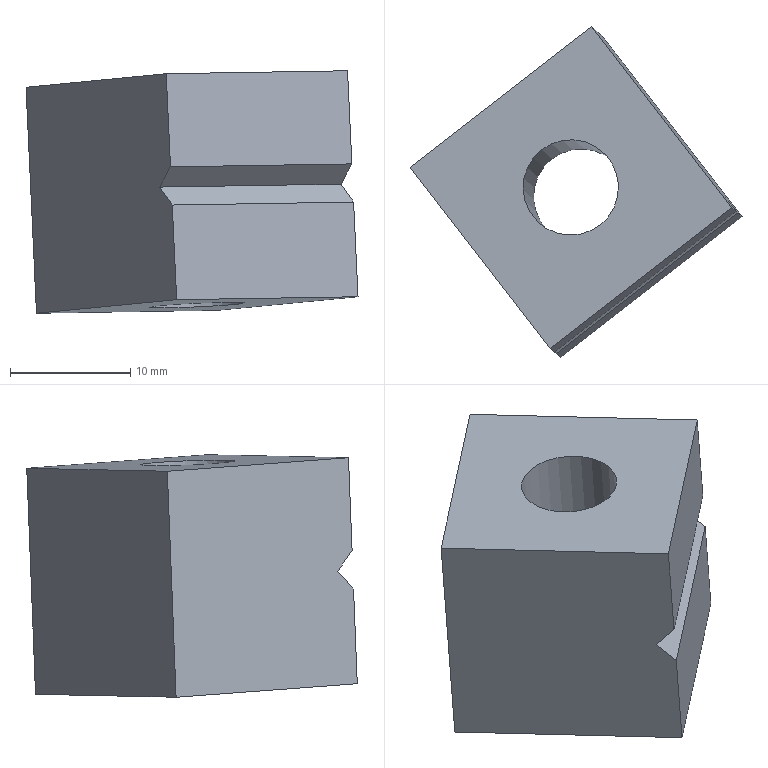Component | NX | MORDAZA_A | 1 solid | 10 faces | box 27.56 x 27.44 x 20.13 mm | volume 5846 mm3 | plane 9 | cylinder 1 | commonest cylinder face diameters 7.925 x1
STEP:
#1=CARTESIAN_POINT('',(0.,0.,0.));
#2=DIRECTION('',(0.,0.,1.));
#3=DIRECTION('',(1.,0.,0.));
#4=AXIS2_PLACEMENT_3D('',#1,#2,#3);
#5=CARTESIAN_POINT('',(8.274,15.453,4.593));
#6=VERTEX_POINT('',#5);
#7=CARTESIAN_POINT('',(-6.781,3.784,4.349));
#8=VERTEX_POINT('',#7);
#9=CARTESIAN_POINT('',(14.096,19.966,4.687));
#10=DIRECTION('',(-0.7903,-0.6126,-0.0128));
#11=VECTOR('',#10,1.);
#12=LINE('',#9,#11);
#13=CARTESIAN_POINT('',(-7.139,4.084,12.082));
#14=DIRECTION('',(-0.611,0.7895,-0.059));
#15=DIRECTION('',(-0.04625,0.03881,0.9982));
#16=AXIS2_PLACEMENT_3D('',#13,#14,#15);
#17=PLANE('',#16);
#18=CARTESIAN_POINT('',(-7.747,26.416));
#19=DIRECTION('',(-0.,-1.));
#20=VECTOR('',#19,1.);
#21=LINE('',#18,#20);
#22=(GEOMETRIC_REPRESENTATION_CONTEXT(2)PARAMETRIC_REPRESENTATION_CONTEXT()REPRESENTATION_CONTEXT('',''));
#23=DEFINITIONAL_REPRESENTATION('',(#21),#22);
#24=PCURVE('',#17,#23);
#25=CARTESIAN_POINT('',(14.096,19.966,4.687));
#26=DIRECTION('',(-0.4647,0.5857,0.6641));
#27=DIRECTION('',(0.3993,-0.5308,0.7475));
#28=AXIS2_PLACEMENT_3D('',#25,#26,#27);
#29=PLANE('',#28);
#30=CARTESIAN_POINT('',(0.,0.));
#31=DIRECTION('',(-0.,-1.));
#32=VECTOR('',#31,1.);
#33=LINE('',#30,#32);
#34=(GEOMETRIC_REPRESENTATION_CONTEXT(2)PARAMETRIC_REPRESENTATION_CONTEXT()REPRESENTATION_CONTEXT('',''));
#35=DEFINITIONAL_REPRESENTATION('',(#33),#34);
#36=PCURVE('',#29,#35);
#37=SURFACE_CURVE('',#12,(#24,#36),.PCURVE_S1.);
#38=EDGE_CURVE('',#6,#8,#37,.T.);
#39=ORIENTED_EDGE('',*,*,#38,.F.);
#40=CARTESIAN_POINT('',(7.916,15.754,12.325));
#41=VERTEX_POINT('',#40);
#42=CARTESIAN_POINT('',(7.916,15.754,12.325));
#43=DIRECTION('',(0.04625,-0.03881,-0.9982));
#44=VECTOR('',#43,1.);
#45=LINE('',#42,#44);
#46=CARTESIAN_POINT('',(0.,19.05));
#47=DIRECTION('',(-1.,0.));
#48=VECTOR('',#47,1.);
#49=LINE('',#46,#48);
#50=(GEOMETRIC_REPRESENTATION_CONTEXT(2)PARAMETRIC_REPRESENTATION_CONTEXT()REPRESENTATION_CONTEXT('',''));
#51=DEFINITIONAL_REPRESENTATION('',(#49),#50);
#52=PCURVE('',#17,#51);
#53=CARTESIAN_POINT('',(7.916,15.754,12.325));
#54=DIRECTION('',(-0.7903,-0.6126,-0.0128));
#55=DIRECTION('',(0.04625,-0.03881,-0.9982));
#56=AXIS2_PLACEMENT_3D('',#53,#54,#55);
#57=PLANE('',#56);
#58=CARTESIAN_POINT('',(0.,0.));
#59=DIRECTION('',(1.,-0.));
#60=VECTOR('',#59,1.);
#61=LINE('',#58,#60);
#62=(GEOMETRIC_REPRESENTATION_CONTEXT(2)PARAMETRIC_REPRESENTATION_CONTEXT()REPRESENTATION_CONTEXT('',''));
#63=DEFINITIONAL_REPRESENTATION('',(#61),#62);
#64=PCURVE('',#57,#63);
#65=SURFACE_CURVE('',#45,(#52,#64),.PCURVE_S1.);
#66=EDGE_CURVE('',#41,#6,#65,.T.);
#67=ORIENTED_EDGE('',*,*,#66,.F.);
#68=CARTESIAN_POINT('',(-7.139,4.084,12.082));
#69=VERTEX_POINT('',#68);
#70=CARTESIAN_POINT('',(-7.139,4.084,12.082));
#71=DIRECTION('',(0.7903,0.6126,0.0128));
#72=VECTOR('',#71,1.);
#73=LINE('',#70,#72);
#74=CARTESIAN_POINT('',(0.,0.));
#75=DIRECTION('',(0.,1.));
#76=VECTOR('',#75,1.);
#77=LINE('',#74,#76);
#78=(GEOMETRIC_REPRESENTATION_CONTEXT(2)PARAMETRIC_REPRESENTATION_CONTEXT()REPRESENTATION_CONTEXT('',''));
#79=DEFINITIONAL_REPRESENTATION('',(#77),#78);
#80=PCURVE('',#17,#79);
#81=CARTESIAN_POINT('',(-18.778,19.124,10.958));
#82=DIRECTION('',(-0.04625,0.03881,0.9982));
#83=DIRECTION('',(0.611,-0.7895,0.059));
#84=AXIS2_PLACEMENT_3D('',#81,#82,#83);
#85=PLANE('',#84);
#86=CARTESIAN_POINT('',(19.05,-0.));
#87=DIRECTION('',(0.,1.));
#88=VECTOR('',#87,1.);
#89=LINE('',#86,#88);
#90=(GEOMETRIC_REPRESENTATION_CONTEXT(2)PARAMETRIC_REPRESENTATION_CONTEXT()REPRESENTATION_CONTEXT('',''));
#91=DEFINITIONAL_REPRESENTATION('',(#89),#90);
#92=PCURVE('',#85,#91);
#93=SURFACE_CURVE('',#73,(#80,#92),.PCURVE_S1.);
#94=EDGE_CURVE('',#69,#41,#93,.T.);
#95=ORIENTED_EDGE('',*,*,#94,.F.);
#96=CARTESIAN_POINT('',(-7.139,4.084,12.082));
#97=DIRECTION('',(0.04625,-0.03881,-0.9982));
#98=VECTOR('',#97,1.);
#99=LINE('',#96,#98);
#100=CARTESIAN_POINT('',(0.,0.));
#101=DIRECTION('',(-1.,0.));
#102=VECTOR('',#101,1.);
#103=LINE('',#100,#102);
#104=(GEOMETRIC_REPRESENTATION_CONTEXT(2)PARAMETRIC_REPRESENTATION_CONTEXT()REPRESENTATION_CONTEXT('',''));
#105=DEFINITIONAL_REPRESENTATION('',(#103),#104);
#106=PCURVE('',#17,#105);
#107=CARTESIAN_POINT('',(-18.778,19.124,10.958));
#108=DIRECTION('',(0.7903,0.6126,0.0128));
#109=DIRECTION('',(-0.04625,0.03881,0.9982));
#110=AXIS2_PLACEMENT_3D('',#107,#108,#109);
#111=PLANE('',#110);
#112=CARTESIAN_POINT('',(-0.,19.05));
#113=DIRECTION('',(-1.,-0.));
#114=VECTOR('',#113,1.);
#115=LINE('',#112,#114);
#116=(GEOMETRIC_REPRESENTATION_CONTEXT(2)PARAMETRIC_REPRESENTATION_CONTEXT()REPRESENTATION_CONTEXT('',''));
#117=DEFINITIONAL_REPRESENTATION('',(#115),#116);
#118=PCURVE('',#111,#117);
#119=SURFACE_CURVE('',#99,(#106,#118),.PCURVE_S1.);
#120=EDGE_CURVE('',#69,#8,#119,.T.);
#121=ORIENTED_EDGE('',*,*,#120,.T.);
#122=EDGE_LOOP('',(#39,#67,#95,#121));
#123=FACE_BOUND('',#122,.T.);
#124=ADVANCED_FACE('',(#123),#17,.F.);
#125=CARTESIAN_POINT('',(-2.853,30.064,-7.56));
#126=VERTEX_POINT('',#125);
#127=CARTESIAN_POINT('',(-17.909,18.394,-7.804));
#128=VERTEX_POINT('',#127);
#129=CARTESIAN_POINT('',(-2.853,30.064,-7.56));
#130=DIRECTION('',(-0.7903,-0.6126,-0.0128));
#131=VECTOR('',#130,1.);
#132=LINE('',#129,#131);
#133=CARTESIAN_POINT('',(-3.723,30.793,11.202));
#134=DIRECTION('',(0.611,-0.7895,0.059));
#135=DIRECTION('',(0.04625,-0.03881,-0.9982));
#136=AXIS2_PLACEMENT_3D('',#133,#134,#135);
#137=PLANE('',#136);
#138=CARTESIAN_POINT('',(18.796,0.));
#139=DIRECTION('',(0.,-1.));
#140=VECTOR('',#139,1.);
#141=LINE('',#138,#140);
#142=(GEOMETRIC_REPRESENTATION_CONTEXT(2)PARAMETRIC_REPRESENTATION_CONTEXT()REPRESENTATION_CONTEXT('',''));
#143=DEFINITIONAL_REPRESENTATION('',(#141),#142);
#144=PCURVE('',#137,#143);
#145=CARTESIAN_POINT('',(-17.909,18.394,-7.804));
#146=DIRECTION('',(-0.04625,0.03881,0.9982));
#147=DIRECTION('',(0.611,-0.7895,0.059));
#148=AXIS2_PLACEMENT_3D('',#145,#146,#147);
#149=PLANE('',#148);
#150=CARTESIAN_POINT('',(-0.,19.05));
#151=DIRECTION('',(-0.,-1.));
#152=VECTOR('',#151,1.);
#153=LINE('',#150,#152);
#154=(GEOMETRIC_REPRESENTATION_CONTEXT(2)PARAMETRIC_REPRESENTATION_CONTEXT()REPRESENTATION_CONTEXT('',''));
#155=DEFINITIONAL_REPRESENTATION('',(#153),#154);
#156=PCURVE('',#149,#155);
#157=SURFACE_CURVE('',#132,(#144,#156),.PCURVE_S1.);
#158=EDGE_CURVE('',#126,#128,#157,.T.);
#159=ORIENTED_EDGE('',*,*,#158,.T.);
#160=CARTESIAN_POINT('',(-18.778,19.124,10.958));
#161=VERTEX_POINT('',#160);
#162=CARTESIAN_POINT('',(-18.778,19.124,10.958));
#163=DIRECTION('',(0.04625,-0.03881,-0.9982));
#164=VECTOR('',#163,1.);
#165=LINE('',#162,#164);
#166=CARTESIAN_POINT('',(-0.,-19.05));
#167=DIRECTION('',(1.,0.));
#168=VECTOR('',#167,1.);
#169=LINE('',#166,#168);
#170=(GEOMETRIC_REPRESENTATION_CONTEXT(2)PARAMETRIC_REPRESENTATION_CONTEXT()REPRESENTATION_CONTEXT('',''));
#171=DEFINITIONAL_REPRESENTATION('',(#169),#170);
#172=PCURVE('',#137,#171);
#173=CARTESIAN_POINT('',(0.,0.));
#174=DIRECTION('',(-1.,-0.));
#175=VECTOR('',#174,1.);
#176=LINE('',#173,#175);
#177=(GEOMETRIC_REPRESENTATION_CONTEXT(2)PARAMETRIC_REPRESENTATION_CONTEXT()REPRESENTATION_CONTEXT('',''));
#178=DEFINITIONAL_REPRESENTATION('',(#176),#177);
#179=PCURVE('',#111,#178);
#180=SURFACE_CURVE('',#165,(#172,#179),.PCURVE_S1.);
#181=EDGE_CURVE('',#161,#128,#180,.T.);
#182=ORIENTED_EDGE('',*,*,#181,.F.);
#183=CARTESIAN_POINT('',(-3.723,30.793,11.202));
#184=VERTEX_POINT('',#183);
#185=CARTESIAN_POINT('',(-3.723,30.793,11.202));
#186=DIRECTION('',(-0.7903,-0.6126,-0.0128));
#187=VECTOR('',#186,1.);
#188=LINE('',#185,#187);
#189=CARTESIAN_POINT('',(0.,0.));
#190=DIRECTION('',(0.,-1.));
#191=VECTOR('',#190,1.);
#192=LINE('',#189,#191);
#193=(GEOMETRIC_REPRESENTATION_CONTEXT(2)PARAMETRIC_REPRESENTATION_CONTEXT()REPRESENTATION_CONTEXT('',''));
#194=DEFINITIONAL_REPRESENTATION('',(#192),#193);
#195=PCURVE('',#137,#194);
#196=CARTESIAN_POINT('',(0.,19.05));
#197=DIRECTION('',(-0.,-1.));
#198=VECTOR('',#197,1.);
#199=LINE('',#196,#198);
#200=(GEOMETRIC_REPRESENTATION_CONTEXT(2)PARAMETRIC_REPRESENTATION_CONTEXT()REPRESENTATION_CONTEXT('',''));
#201=DEFINITIONAL_REPRESENTATION('',(#199),#200);
#202=PCURVE('',#85,#201);
#203=SURFACE_CURVE('',#188,(#195,#202),.PCURVE_S1.);
#204=EDGE_CURVE('',#184,#161,#203,.T.);
#205=ORIENTED_EDGE('',*,*,#204,.F.);
#206=CARTESIAN_POINT('',(-3.723,30.793,11.202));
#207=DIRECTION('',(0.04625,-0.03881,-0.9982));
#208=VECTOR('',#207,1.);
#209=LINE('',#206,#208);
#210=CARTESIAN_POINT('',(0.,0.));
#211=DIRECTION('',(1.,0.));
#212=VECTOR('',#211,1.);
#213=LINE('',#210,#212);
#214=(GEOMETRIC_REPRESENTATION_CONTEXT(2)PARAMETRIC_REPRESENTATION_CONTEXT()REPRESENTATION_CONTEXT('',''));
#215=DEFINITIONAL_REPRESENTATION('',(#213),#214);
#216=PCURVE('',#137,#215);
#217=CARTESIAN_POINT('',(-0.,-19.05));
#218=DIRECTION('',(1.,-0.));
#219=VECTOR('',#218,1.);
#220=LINE('',#217,#219);
#221=(GEOMETRIC_REPRESENTATION_CONTEXT(2)PARAMETRIC_REPRESENTATION_CONTEXT()REPRESENTATION_CONTEXT('',''));
#222=DEFINITIONAL_REPRESENTATION('',(#220),#221);
#223=PCURVE('',#57,#222);
#224=SURFACE_CURVE('',#209,(#216,#223),.PCURVE_S1.);
#225=EDGE_CURVE('',#184,#126,#224,.T.);
#226=ORIENTED_EDGE('',*,*,#225,.T.);
#227=EDGE_LOOP('',(#159,#182,#205,#226));
#228=FACE_BOUND('',#227,.T.);
#229=ADVANCED_FACE('',(#228),#137,.F.);
#230=CARTESIAN_POINT('',(-6.634,3.661,1.18));
#231=VERTEX_POINT('',#230);
#232=CARTESIAN_POINT('',(-6.27,3.355,-6.68));
#233=VERTEX_POINT('',#232);
#234=CARTESIAN_POINT('',(-7.139,4.084,12.082));
#235=DIRECTION('',(0.04625,-0.03881,-0.9982));
#236=VECTOR('',#235,1.);
#237=LINE('',#234,#236);
#238=CARTESIAN_POINT('',(-0.,19.05));
#239=DIRECTION('',(-1.,-0.));
#240=VECTOR('',#239,1.);
#241=LINE('',#238,#240);
#242=(GEOMETRIC_REPRESENTATION_CONTEXT(2)PARAMETRIC_REPRESENTATION_CONTEXT()REPRESENTATION_CONTEXT('',''));
#243=DEFINITIONAL_REPRESENTATION('',(#241),#242);
#244=PCURVE('',#111,#243);
#245=CARTESIAN_POINT('',(-7.139,4.084,12.082));
#246=DIRECTION('',(-0.611,0.7895,-0.059));
#247=DIRECTION('',(-0.04625,0.03881,0.9982));
#248=AXIS2_PLACEMENT_3D('',#245,#246,#247);
#249=PLANE('',#248);
#250=CARTESIAN_POINT('',(0.,0.));
#251=DIRECTION('',(-1.,0.));
#252=VECTOR('',#251,1.);
#253=LINE('',#250,#252);
#254=(GEOMETRIC_REPRESENTATION_CONTEXT(2)PARAMETRIC_REPRESENTATION_CONTEXT()REPRESENTATION_CONTEXT('',''));
#255=DEFINITIONAL_REPRESENTATION('',(#253),#254);
#256=PCURVE('',#249,#255);
#257=SURFACE_CURVE('',#237,(#244,#256),.PCURVE_S1.);
#258=EDGE_CURVE('',#231,#233,#257,.T.);
#259=ORIENTED_EDGE('',*,*,#258,.F.);
#260=CARTESIAN_POINT('',(-7.677,4.975,2.67));
#261=VERTEX_POINT('',#260);
#262=CARTESIAN_POINT('',(-16.483,16.073,15.254));
#263=DIRECTION('',(-0.4647,0.5857,0.6641));
#264=VECTOR('',#263,1.);
#265=LINE('',#262,#264);
#266=CARTESIAN_POINT('',(4.064,4.064));
#267=DIRECTION('',(0.7071,-0.7071));
#268=VECTOR('',#267,1.);
#269=LINE('',#266,#268);
#270=(GEOMETRIC_REPRESENTATION_CONTEXT(2)PARAMETRIC_REPRESENTATION_CONTEXT()REPRESENTATION_CONTEXT('',''));
#271=DEFINITIONAL_REPRESENTATION('',(#269),#270);
#272=PCURVE('',#111,#271);
#273=CARTESIAN_POINT('',(13.199,21.157,3.009));
#274=DIRECTION('',(-0.3993,0.5308,-0.7475));
#275=DIRECTION('',(-0.4647,0.5857,0.6641));
#276=AXIS2_PLACEMENT_3D('',#273,#274,#275);
#277=PLANE('',#276);
#278=CARTESIAN_POINT('',(18.948,-26.416));
#279=DIRECTION('',(1.,0.));
#280=VECTOR('',#279,1.);
#281=LINE('',#278,#280);
#282=(GEOMETRIC_REPRESENTATION_CONTEXT(2)PARAMETRIC_REPRESENTATION_CONTEXT()REPRESENTATION_CONTEXT('',''));
#283=DEFINITIONAL_REPRESENTATION('',(#281),#282);
#284=PCURVE('',#277,#283);
#285=SURFACE_CURVE('',#265,(#272,#284),.PCURVE_S1.);
#286=EDGE_CURVE('',#231,#261,#285,.T.);
#287=ORIENTED_EDGE('',*,*,#286,.T.);
#288=CARTESIAN_POINT('',(-9.972,8.026,-1.626));
#289=DIRECTION('',(0.3993,-0.5308,0.7475));
#290=VECTOR('',#289,1.);
#291=LINE('',#288,#290);
#292=CARTESIAN_POINT('',(-13.399,13.399));
#293=DIRECTION('',(0.7071,0.7071));
#294=VECTOR('',#293,1.);
#295=LINE('',#292,#294);
#296=(GEOMETRIC_REPRESENTATION_CONTEXT(2)PARAMETRIC_REPRESENTATION_CONTEXT()REPRESENTATION_CONTEXT('',''));
#297=DEFINITIONAL_REPRESENTATION('',(#295),#296);
#298=PCURVE('',#111,#297);
#299=CARTESIAN_POINT('',(-7.992,-26.416));
#300=DIRECTION('',(1.,0.));
#301=VECTOR('',#300,1.);
#302=LINE('',#299,#301);
#303=(GEOMETRIC_REPRESENTATION_CONTEXT(2)PARAMETRIC_REPRESENTATION_CONTEXT()REPRESENTATION_CONTEXT('',''));
#304=DEFINITIONAL_REPRESENTATION('',(#302),#303);
#305=PCURVE('',#29,#304);
#306=SURFACE_CURVE('',#291,(#298,#305),.PCURVE_S1.);
#307=EDGE_CURVE('',#261,#8,#306,.T.);
#308=ORIENTED_EDGE('',*,*,#307,.T.);
#309=ORIENTED_EDGE('',*,*,#120,.F.);
#310=CARTESIAN_POINT('',(-18.778,19.124,10.958));
#311=DIRECTION('',(0.611,-0.7895,0.059));
#312=VECTOR('',#311,1.);
#313=LINE('',#310,#312);
#314=CARTESIAN_POINT('',(0.,0.));
#315=DIRECTION('',(-0.,1.));
#316=VECTOR('',#315,1.);
#317=LINE('',#314,#316);
#318=(GEOMETRIC_REPRESENTATION_CONTEXT(2)PARAMETRIC_REPRESENTATION_CONTEXT()REPRESENTATION_CONTEXT('',''));
#319=DEFINITIONAL_REPRESENTATION('',(#317),#318);
#320=PCURVE('',#111,#319);
#321=CARTESIAN_POINT('',(0.,0.));
#322=DIRECTION('',(1.,-0.));
#323=VECTOR('',#322,1.);
#324=LINE('',#321,#323);
#325=(GEOMETRIC_REPRESENTATION_CONTEXT(2)PARAMETRIC_REPRESENTATION_CONTEXT()REPRESENTATION_CONTEXT('',''));
#326=DEFINITIONAL_REPRESENTATION('',(#324),#325);
#327=PCURVE('',#85,#326);
#328=SURFACE_CURVE('',#313,(#320,#327),.PCURVE_S1.);
#329=EDGE_CURVE('',#161,#69,#328,.T.);
#330=ORIENTED_EDGE('',*,*,#329,.F.);
#331=ORIENTED_EDGE('',*,*,#181,.T.);
#332=CARTESIAN_POINT('',(-17.909,18.394,-7.804));
#333=DIRECTION('',(0.611,-0.7895,0.059));
#334=VECTOR('',#333,1.);
#335=LINE('',#332,#334);
#336=CARTESIAN_POINT('',(-18.796,-0.));
#337=DIRECTION('',(-0.,1.));
#338=VECTOR('',#337,1.);
#339=LINE('',#336,#338);
#340=(GEOMETRIC_REPRESENTATION_CONTEXT(2)PARAMETRIC_REPRESENTATION_CONTEXT()REPRESENTATION_CONTEXT('',''));
#341=DEFINITIONAL_REPRESENTATION('',(#339),#340);
#342=PCURVE('',#111,#341);
#343=CARTESIAN_POINT('',(0.,0.));
#344=DIRECTION('',(1.,-0.));
#345=VECTOR('',#344,1.);
#346=LINE('',#343,#345);
#347=(GEOMETRIC_REPRESENTATION_CONTEXT(2)PARAMETRIC_REPRESENTATION_CONTEXT()REPRESENTATION_CONTEXT('',''));
#348=DEFINITIONAL_REPRESENTATION('',(#346),#347);
#349=PCURVE('',#149,#348);
#350=SURFACE_CURVE('',#335,(#342,#349),.PCURVE_S1.);
#351=EDGE_CURVE('',#128,#233,#350,.T.);
#352=ORIENTED_EDGE('',*,*,#351,.T.);
#353=EDGE_LOOP('',(#259,#287,#308,#309,#330,#331,#352));
#354=FACE_BOUND('',#353,.T.);
#355=ADVANCED_FACE('',(#354),#111,.F.);
#356=CARTESIAN_POINT('',(8.421,15.33,1.423));
#357=VERTEX_POINT('',#356);
#358=CARTESIAN_POINT('',(8.785,15.025,-6.436));
#359=VERTEX_POINT('',#358);
#360=CARTESIAN_POINT('',(7.916,15.754,12.325));
#361=DIRECTION('',(0.04625,-0.03881,-0.9982));
#362=VECTOR('',#361,1.);
#363=LINE('',#360,#362);
#364=CARTESIAN_POINT('',(0.,19.05));
#365=DIRECTION('',(-1.,0.));
#366=VECTOR('',#365,1.);
#367=LINE('',#364,#366);
#368=(GEOMETRIC_REPRESENTATION_CONTEXT(2)PARAMETRIC_REPRESENTATION_CONTEXT()REPRESENTATION_CONTEXT('',''));
#369=DEFINITIONAL_REPRESENTATION('',(#367),#368);
#370=PCURVE('',#249,#369);
#371=CARTESIAN_POINT('',(0.,0.));
#372=DIRECTION('',(1.,-0.));
#373=VECTOR('',#372,1.);
#374=LINE('',#371,#373);
#375=(GEOMETRIC_REPRESENTATION_CONTEXT(2)PARAMETRIC_REPRESENTATION_CONTEXT()REPRESENTATION_CONTEXT('',''));
#376=DEFINITIONAL_REPRESENTATION('',(#374),#375);
#377=PCURVE('',#57,#376);
#378=SURFACE_CURVE('',#363,(#370,#377),.PCURVE_S1.);
#379=EDGE_CURVE('',#357,#359,#378,.T.);
#380=ORIENTED_EDGE('',*,*,#379,.F.);
#381=CARTESIAN_POINT('',(14.243,19.842,1.518));
#382=DIRECTION('',(-0.7903,-0.6126,-0.0128));
#383=VECTOR('',#382,1.);
#384=LINE('',#381,#383);
#385=CARTESIAN_POINT('',(-10.922,26.416));
#386=DIRECTION('',(-0.,-1.));
#387=VECTOR('',#386,1.);
#388=LINE('',#385,#387);
#389=(GEOMETRIC_REPRESENTATION_CONTEXT(2)PARAMETRIC_REPRESENTATION_CONTEXT()REPRESENTATION_CONTEXT('',''));
#390=DEFINITIONAL_REPRESENTATION('',(#388),#389);
#391=PCURVE('',#249,#390);
#392=CARTESIAN_POINT('',(-2.245,0.));
#393=DIRECTION('',(-0.,-1.));
#394=VECTOR('',#393,1.);
#395=LINE('',#392,#394);
#396=(GEOMETRIC_REPRESENTATION_CONTEXT(2)PARAMETRIC_REPRESENTATION_CONTEXT()REPRESENTATION_CONTEXT('',''));
#397=DEFINITIONAL_REPRESENTATION('',(#395),#396);
#398=PCURVE('',#277,#397);
#399=SURFACE_CURVE('',#384,(#391,#398),.PCURVE_S1.);
#400=EDGE_CURVE('',#357,#231,#399,.T.);
#401=ORIENTED_EDGE('',*,*,#400,.T.);
#402=ORIENTED_EDGE('',*,*,#258,.T.);
#403=CARTESIAN_POINT('',(-6.27,3.355,-6.68));
#404=DIRECTION('',(0.7903,0.6126,0.0128));
#405=VECTOR('',#404,1.);
#406=LINE('',#403,#405);
#407=CARTESIAN_POINT('',(-18.796,0.));
#408=DIRECTION('',(0.,1.));
#409=VECTOR('',#408,1.);
#410=LINE('',#407,#409);
#411=(GEOMETRIC_REPRESENTATION_CONTEXT(2)PARAMETRIC_REPRESENTATION_CONTEXT()REPRESENTATION_CONTEXT('',''));
#412=DEFINITIONAL_REPRESENTATION('',(#410),#411);
#413=PCURVE('',#249,#412);
#414=CARTESIAN_POINT('',(19.05,0.));
#415=DIRECTION('',(0.,1.));
#416=VECTOR('',#415,1.);
#417=LINE('',#414,#416);
#418=(GEOMETRIC_REPRESENTATION_CONTEXT(2)PARAMETRIC_REPRESENTATION_CONTEXT()REPRESENTATION_CONTEXT('',''));
#419=DEFINITIONAL_REPRESENTATION('',(#417),#418);
#420=PCURVE('',#149,#419);
#421=SURFACE_CURVE('',#406,(#413,#420),.PCURVE_S1.);
#422=EDGE_CURVE('',#233,#359,#421,.T.);
#423=ORIENTED_EDGE('',*,*,#422,.T.);
#424=EDGE_LOOP('',(#380,#401,#402,#423));
#425=FACE_BOUND('',#424,.T.);
#426=ADVANCED_FACE('',(#425),#249,.F.);
#427=CARTESIAN_POINT('',(7.378,16.645,2.914));
#428=VERTEX_POINT('',#427);
#429=CARTESIAN_POINT('',(10.462,12.546,8.688));
#430=DIRECTION('',(-0.3993,0.5308,-0.7475));
#431=VECTOR('',#430,1.);
#432=LINE('',#429,#431);
#433=CARTESIAN_POINT('',(3.873,3.873));
#434=DIRECTION('',(0.7071,-0.7071));
#435=VECTOR('',#434,1.);
#436=LINE('',#433,#435);
#437=(GEOMETRIC_REPRESENTATION_CONTEXT(2)PARAMETRIC_REPRESENTATION_CONTEXT()REPRESENTATION_CONTEXT('',''));
#438=DEFINITIONAL_REPRESENTATION('',(#436),#437);
#439=PCURVE('',#57,#438);
#440=CARTESIAN_POINT('',(5.478,-7.366));
#441=DIRECTION('',(-1.,-0.));
#442=VECTOR('',#441,1.);
#443=LINE('',#440,#442);
#444=(GEOMETRIC_REPRESENTATION_CONTEXT(2)PARAMETRIC_REPRESENTATION_CONTEXT()REPRESENTATION_CONTEXT('',''));
#445=DEFINITIONAL_REPRESENTATION('',(#443),#444);
#446=PCURVE('',#29,#445);
#447=SURFACE_CURVE('',#432,(#439,#446),.PCURVE_S1.);
#448=EDGE_CURVE('',#6,#428,#447,.T.);
#449=ORIENTED_EDGE('',*,*,#448,.T.);
#450=CARTESIAN_POINT('',(4.832,19.853,6.552));
#451=DIRECTION('',(0.4647,-0.5857,-0.6641));
#452=VECTOR('',#451,1.);
#453=LINE('',#450,#452);
#454=CARTESIAN_POINT('',(5.461,-5.461));
#455=DIRECTION('',(0.7071,0.7071));
#456=VECTOR('',#455,1.);
#457=LINE('',#454,#456);
#458=(GEOMETRIC_REPRESENTATION_CONTEXT(2)PARAMETRIC_REPRESENTATION_CONTEXT()REPRESENTATION_CONTEXT('',''));
#459=DEFINITIONAL_REPRESENTATION('',(#457),#458);
#460=PCURVE('',#57,#459);
#461=CARTESIAN_POINT('',(5.478,-7.366));
#462=DIRECTION('',(-1.,-0.));
#463=VECTOR('',#462,1.);
#464=LINE('',#461,#463);
#465=(GEOMETRIC_REPRESENTATION_CONTEXT(2)PARAMETRIC_REPRESENTATION_CONTEXT()REPRESENTATION_CONTEXT('',''));
#466=DEFINITIONAL_REPRESENTATION('',(#464),#465);
#467=PCURVE('',#277,#466);
#468=SURFACE_CURVE('',#453,(#460,#467),.PCURVE_S1.);
#469=EDGE_CURVE('',#428,#357,#468,.T.);
#470=ORIENTED_EDGE('',*,*,#469,.T.);
#471=ORIENTED_EDGE('',*,*,#379,.T.);
#472=CARTESIAN_POINT('',(8.785,15.025,-6.436));
#473=DIRECTION('',(-0.611,0.7895,-0.059));
#474=VECTOR('',#473,1.);
#475=LINE('',#472,#474);
#476=CARTESIAN_POINT('',(18.796,0.));
#477=DIRECTION('',(-0.,-1.));
#478=VECTOR('',#477,1.);
#479=LINE('',#476,#478);
#480=(GEOMETRIC_REPRESENTATION_CONTEXT(2)PARAMETRIC_REPRESENTATION_CONTEXT()REPRESENTATION_CONTEXT('',''));
#481=DEFINITIONAL_REPRESENTATION('',(#479),#480);
#482=PCURVE('',#57,#481);
#483=CARTESIAN_POINT('',(19.05,19.05));
#484=DIRECTION('',(-1.,0.));
#485=VECTOR('',#484,1.);
#486=LINE('',#483,#485);
#487=(GEOMETRIC_REPRESENTATION_CONTEXT(2)PARAMETRIC_REPRESENTATION_CONTEXT()REPRESENTATION_CONTEXT('',''));
#488=DEFINITIONAL_REPRESENTATION('',(#486),#487);
#489=PCURVE('',#149,#488);
#490=SURFACE_CURVE('',#475,(#482,#489),.PCURVE_S1.);
#491=EDGE_CURVE('',#359,#126,#490,.T.);
#492=ORIENTED_EDGE('',*,*,#491,.T.);
#493=ORIENTED_EDGE('',*,*,#225,.F.);
#494=CARTESIAN_POINT('',(7.916,15.754,12.325));
#495=DIRECTION('',(-0.611,0.7895,-0.059));
#496=VECTOR('',#495,1.);
#497=LINE('',#494,#496);
#498=CARTESIAN_POINT('',(0.,0.));
#499=DIRECTION('',(-0.,-1.));
#500=VECTOR('',#499,1.);
#501=LINE('',#498,#500);
#502=(GEOMETRIC_REPRESENTATION_CONTEXT(2)PARAMETRIC_REPRESENTATION_CONTEXT()REPRESENTATION_CONTEXT('',''));
#503=DEFINITIONAL_REPRESENTATION('',(#501),#502);
#504=PCURVE('',#57,#503);
#505=CARTESIAN_POINT('',(19.05,19.05));
#506=DIRECTION('',(-1.,0.));
#507=VECTOR('',#506,1.);
#508=LINE('',#505,#507);
#509=(GEOMETRIC_REPRESENTATION_CONTEXT(2)PARAMETRIC_REPRESENTATION_CONTEXT()REPRESENTATION_CONTEXT('',''));
#510=DEFINITIONAL_REPRESENTATION('',(#508),#509);
#511=PCURVE('',#85,#510);
#512=SURFACE_CURVE('',#497,(#504,#511),.PCURVE_S1.);
#513=EDGE_CURVE('',#41,#184,#512,.T.);
#514=ORIENTED_EDGE('',*,*,#513,.F.);
#515=ORIENTED_EDGE('',*,*,#66,.T.);
#516=EDGE_LOOP('',(#449,#470,#471,#492,#493,#514,#515));
#517=FACE_BOUND('',#516,.T.);
#518=ADVANCED_FACE('',(#517),#57,.F.);
#519=CARTESIAN_POINT('',(-3.01,14.311,11.875));
#520=VERTEX_POINT('',#519);
#521=CARTESIAN_POINT('',(-5.431,17.439,11.642));
#522=DIRECTION('',(-0.04625,0.03881,0.9982));
#523=DIRECTION('',(0.611,-0.7895,0.059));
#524=AXIS2_PLACEMENT_3D('',#521,#522,#523);
#525=CIRCLE('',#524,3.962);
#526=CARTESIAN_POINT('',(9.525,9.525));
#527=DIRECTION('',(1.,0.));
#528=AXIS2_PLACEMENT_2D('',#526,#527);
#529=CIRCLE('',#528,3.962);
#530=(GEOMETRIC_REPRESENTATION_CONTEXT(2)PARAMETRIC_REPRESENTATION_CONTEXT()REPRESENTATION_CONTEXT('',''));
#531=DEFINITIONAL_REPRESENTATION('',(#529),#530);
#532=PCURVE('',#85,#531);
#533=CARTESIAN_POINT('',(-4.28,16.473,-13.205));
#534=DIRECTION('',(-0.04625,0.03881,0.9982));
#535=DIRECTION('',(0.611,-0.7895,0.059));
#536=AXIS2_PLACEMENT_3D('',#533,#534,#535);
#537=CYLINDRICAL_SURFACE('',#536,3.962);
#538=CARTESIAN_POINT('',(0.,24.892));
#539=DIRECTION('',(1.,0.));
#540=VECTOR('',#539,1.);
#541=LINE('',#538,#540);
#542=(GEOMETRIC_REPRESENTATION_CONTEXT(2)PARAMETRIC_REPRESENTATION_CONTEXT()REPRESENTATION_CONTEXT('',''));
#543=DEFINITIONAL_REPRESENTATION('',(#541),#542);
#544=PCURVE('',#537,#543);
#545=SURFACE_CURVE('',#525,(#532,#544),.PCURVE_S1.);
#546=EDGE_CURVE('',#520,#520,#545,.T.);
#547=ORIENTED_EDGE('',*,*,#546,.F.);
#548=EDGE_LOOP('',(#547));
#549=FACE_BOUND('',#548,.T.);
#550=ORIENTED_EDGE('',*,*,#204,.T.);
#551=ORIENTED_EDGE('',*,*,#329,.T.);
#552=ORIENTED_EDGE('',*,*,#94,.T.);
#553=ORIENTED_EDGE('',*,*,#513,.T.);
#554=EDGE_LOOP('',(#550,#551,#552,#553));
#555=FACE_BOUND('',#554,.T.);
#556=ADVANCED_FACE('',(#549,#555),#85,.T.);
#557=CARTESIAN_POINT('',(-2.141,13.581,-6.886));
#558=VERTEX_POINT('',#557);
#559=CARTESIAN_POINT('',(-4.562,16.709,-7.12));
#560=DIRECTION('',(-0.04625,0.03881,0.9982));
#561=DIRECTION('',(0.611,-0.7895,0.059));
#562=AXIS2_PLACEMENT_3D('',#559,#560,#561);
#563=CIRCLE('',#562,3.962);
#564=CARTESIAN_POINT('',(9.525,9.525));
#565=DIRECTION('',(1.,0.));
#566=AXIS2_PLACEMENT_2D('',#564,#565);
#567=CIRCLE('',#566,3.962);
#568=(GEOMETRIC_REPRESENTATION_CONTEXT(2)PARAMETRIC_REPRESENTATION_CONTEXT()REPRESENTATION_CONTEXT('',''));
#569=DEFINITIONAL_REPRESENTATION('',(#567),#568);
#570=PCURVE('',#149,#569);
#571=CARTESIAN_POINT('',(0.,6.096));
#572=DIRECTION('',(1.,0.));
#573=VECTOR('',#572,1.);
#574=LINE('',#571,#573);
#575=(GEOMETRIC_REPRESENTATION_CONTEXT(2)PARAMETRIC_REPRESENTATION_CONTEXT()REPRESENTATION_CONTEXT('',''));
#576=DEFINITIONAL_REPRESENTATION('',(#574),#575);
#577=PCURVE('',#537,#576);
#578=SURFACE_CURVE('',#563,(#570,#577),.PCURVE_S1.);
#579=EDGE_CURVE('',#558,#558,#578,.T.);
#580=ORIENTED_EDGE('',*,*,#579,.T.);
#581=EDGE_LOOP('',(#580));
#582=FACE_BOUND('',#581,.T.);
#583=ORIENTED_EDGE('',*,*,#158,.F.);
#584=ORIENTED_EDGE('',*,*,#491,.F.);
#585=ORIENTED_EDGE('',*,*,#422,.F.);
#586=ORIENTED_EDGE('',*,*,#351,.F.);
#587=EDGE_LOOP('',(#583,#584,#585,#586));
#588=FACE_BOUND('',#587,.T.);
#589=ADVANCED_FACE('',(#582,#588),#149,.F.);
#590=ORIENTED_EDGE('',*,*,#546,.F.);
#591=CARTESIAN_POINT('',(-2.141,13.581,-6.886));
#592=CARTESIAN_POINT('',(-3.01,14.311,11.875));
#593=B_SPLINE_CURVE_WITH_KNOTS('',1,(#591,#592),.UNSPECIFIED.,.F.,.F.,(2,2),(6.096,24.892),.PIECEWISE_BEZIER_KNOTS.);
#594=CARTESIAN_POINT('',(0.,0.));
#595=DIRECTION('',(0.,1.));
#596=VECTOR('',#595,1.);
#597=LINE('',#594,#596);
#598=(GEOMETRIC_REPRESENTATION_CONTEXT(2)PARAMETRIC_REPRESENTATION_CONTEXT()REPRESENTATION_CONTEXT('',''));
#599=DEFINITIONAL_REPRESENTATION('',(#597),#598);
#600=PCURVE('',#537,#599);
#601=CARTESIAN_POINT('',(6.283,0.));
#602=DIRECTION('',(0.,1.));
#603=VECTOR('',#602,1.);
#604=LINE('',#601,#603);
#605=(GEOMETRIC_REPRESENTATION_CONTEXT(2)PARAMETRIC_REPRESENTATION_CONTEXT()REPRESENTATION_CONTEXT('',''));
#606=DEFINITIONAL_REPRESENTATION('',(#604),#605);
#607=PCURVE('',#537,#606);
#608=SEAM_CURVE('',#593,(#600,#607),.PCURVE_S1.);
#609=EDGE_CURVE('',#558,#520,#608,.T.);
#610=ORIENTED_EDGE('',*,*,#609,.F.);
#611=ORIENTED_EDGE('',*,*,#579,.T.);
#612=ORIENTED_EDGE('',*,*,#609,.T.);
#613=EDGE_LOOP('',(#590,#610,#611,#612));
#614=FACE_BOUND('',#613,.F.);
#615=ADVANCED_FACE('',(#614),#537,.F.);
#616=ORIENTED_EDGE('',*,*,#400,.F.);
#617=ORIENTED_EDGE('',*,*,#469,.F.);
#618=CARTESIAN_POINT('',(13.199,21.157,3.009));
#619=DIRECTION('',(0.7903,0.6126,0.0128));
#620=VECTOR('',#619,1.);
#621=LINE('',#618,#620);
#622=CARTESIAN_POINT('',(0.,0.));
#623=DIRECTION('',(0.,1.));
#624=VECTOR('',#623,1.);
#625=LINE('',#622,#624);
#626=(GEOMETRIC_REPRESENTATION_CONTEXT(2)PARAMETRIC_REPRESENTATION_CONTEXT()REPRESENTATION_CONTEXT('',''));
#627=DEFINITIONAL_REPRESENTATION('',(#625),#626);
#628=PCURVE('',#277,#627);
#629=CARTESIAN_POINT('',(-2.245,0.));
#630=DIRECTION('',(0.,1.));
#631=VECTOR('',#630,1.);
#632=LINE('',#629,#631);
#633=(GEOMETRIC_REPRESENTATION_CONTEXT(2)PARAMETRIC_REPRESENTATION_CONTEXT()REPRESENTATION_CONTEXT('',''));
#634=DEFINITIONAL_REPRESENTATION('',(#632),#633);
#635=PCURVE('',#29,#634);
#636=SURFACE_CURVE('',#621,(#628,#635),.PCURVE_S1.);
#637=EDGE_CURVE('',#261,#428,#636,.T.);
#638=ORIENTED_EDGE('',*,*,#637,.F.);
#639=ORIENTED_EDGE('',*,*,#286,.F.);
#640=EDGE_LOOP('',(#616,#617,#638,#639));
#641=FACE_BOUND('',#640,.T.);
#642=ADVANCED_FACE('',(#641),#277,.F.);
#643=ORIENTED_EDGE('',*,*,#637,.T.);
#644=ORIENTED_EDGE('',*,*,#448,.F.);
#645=ORIENTED_EDGE('',*,*,#38,.T.);
#646=ORIENTED_EDGE('',*,*,#307,.F.);
#647=EDGE_LOOP('',(#643,#644,#645,#646));
#648=FACE_BOUND('',#647,.T.);
#649=ADVANCED_FACE('',(#648),#29,.F.);
#650=CLOSED_SHELL('',(#124,#229,#355,#426,#518,#556,#589,#615,#642,#649));
#651=MANIFOLD_SOLID_BREP('',#650);
#652=(LENGTH_UNIT()NAMED_UNIT(*)SI_UNIT(.MILLI.,.METRE.));
#653=UNCERTAINTY_MEASURE_WITH_UNIT(LENGTH_MEASURE(0.000001),#652,'','');
#654=(NAMED_UNIT(*)PLANE_ANGLE_UNIT()SI_UNIT($,.RADIAN.));
#655=(NAMED_UNIT(*)SI_UNIT($,.STERADIAN.)SOLID_ANGLE_UNIT());
#656=(GEOMETRIC_REPRESENTATION_CONTEXT(3)GLOBAL_UNCERTAINTY_ASSIGNED_CONTEXT((#653))GLOBAL_UNIT_ASSIGNED_CONTEXT((#652,#654,#655))REPRESENTATION_CONTEXT('',''));
#657=ADVANCED_BREP_SHAPE_REPRESENTATION('',(#4,#651),#656);